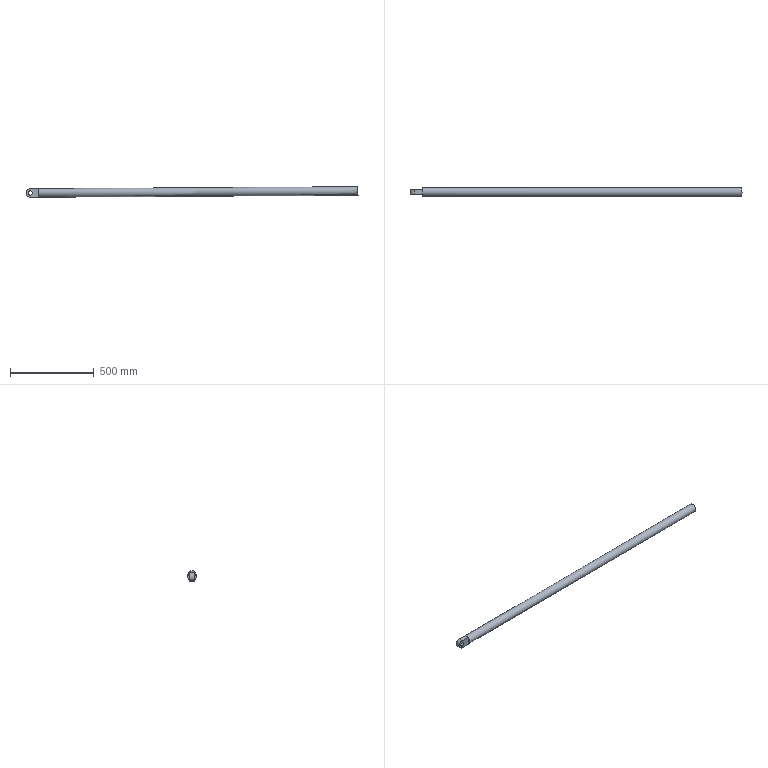Component | NX | MID_ARM_EXT_ROD | 1 solid | 14 faces | volume 3939530 mm3 | plane 11 | cylinder 3 | commonest cylinder face diameters 50.8 x2 25.4 x1